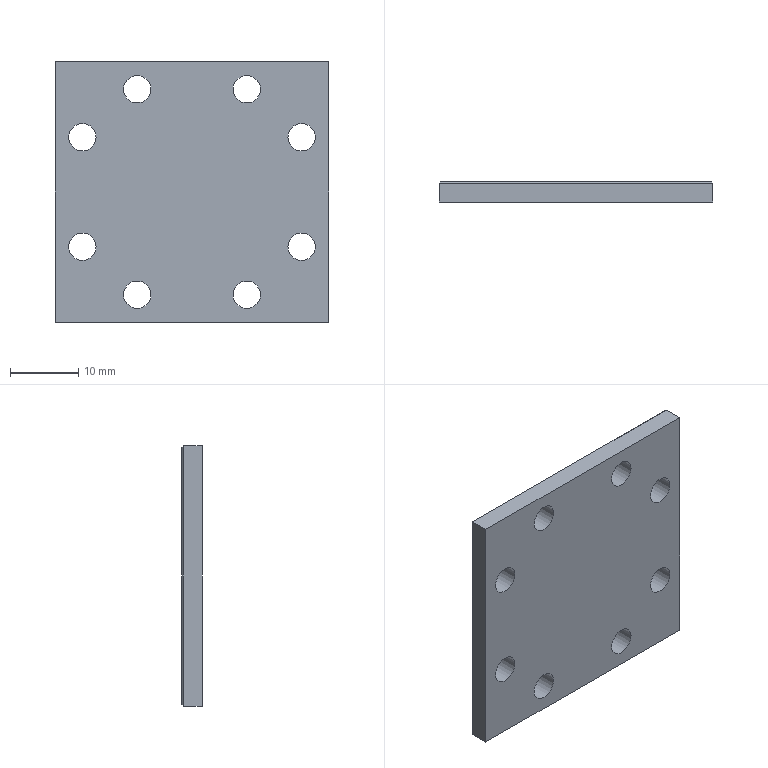Component | NX | EXTERNAL_PISTON_CYLINDER_HEAD | 1 solid | 18 faces | volume 4254 mm3 | plane 10 | cylinder 8 | commonest cylinder face diameters 4 x8